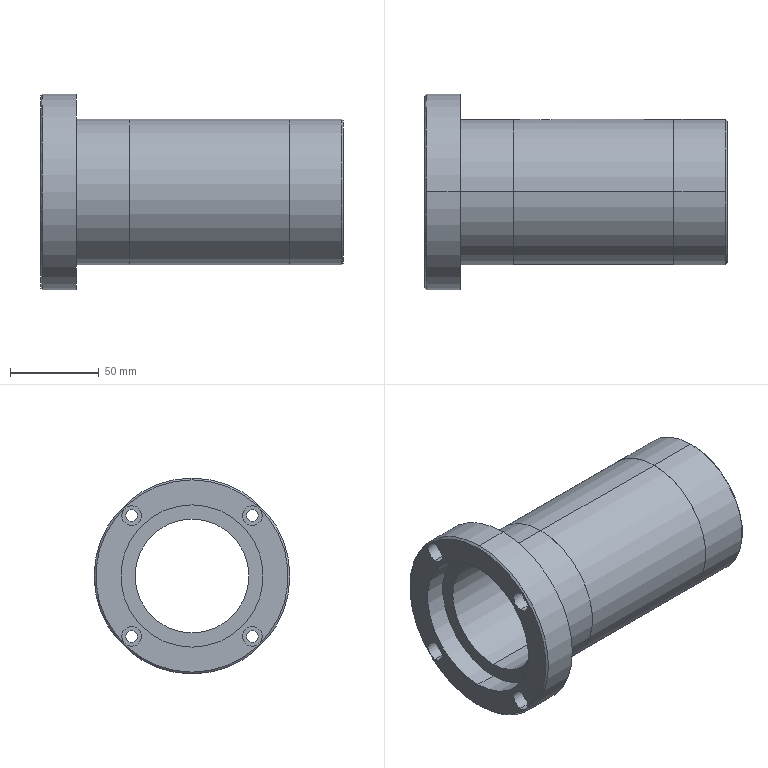Component | SolidWorks | 4-12-12ClampingAxisAssembly-1_4-12-1ClampingTelescopicAxisHousing-1 | 1 solid | 49 faces | box 170 x 110 x 110 mm | volume 405832 mm3 | cylinder 32 | plane 11 | cone 6 | commonest cylinder face diameters 11 x8 6.6 x8 82 x4 10 x2 80 x2 64 x2 81.8 x2 110 x2
build123d program:
from build123d import *

# Parameters (mm, degrees)
HOLE_SIZE_ACCORDING_TO_THE_TYPE_OF_HEX_S_D           = 6.6
HOLE_SIZE_ACCORDING_TO_THE_TYPE_OF_HEX_S_CBORE_D     = 11
HOLE_SIZE_ACCORDING_TO_THE_TYPE_OF_HEX_S_CBORE_DEPTH = 6.8
CIRPATTERN1_COUNT                                    = 4
SKETCH6_W                                            = 4.25
SKETCH6_H                                            = 55
CHAMFER1_SIZE                                        = 1
SKETCH1_R                                            = 5
M10_THREAD_MAJOR_DIAMETER_RELEASE_DEPTH              = 12


with BuildPart() as part:
    # Sketch1_2 → Revolve1 (revolve)
    with BuildSketch(Plane.XY, mode=Mode.PRIVATE) as revolve1_sk:
        Polygon((0, 40), (0, 55), (20, 55), (20, 41), (50, 41), (50, 40.9), (140, 40.9), (140, 41), (170, 41), (170, 32), (12, 32), (12, 40), align=None)
    revolve(revolve1_sk.sketch.rotate(Axis((0, 0, 0), (1, 0, 0)), 90), axis=Axis((0, 0, 0), (1, 0, 0)))

    # Hole Size according to the type of Hex S (through all)
    with Locations(Plane.ZY):
        with Locations((33.941, 33.941)):
            hole_size_according_to_the_type_of_hex_s = CounterBoreHole(HOLE_SIZE_ACCORDING_TO_THE_TYPE_OF_HEX_S_D / 2, HOLE_SIZE_ACCORDING_TO_THE_TYPE_OF_HEX_S_CBORE_D / 2, HOLE_SIZE_ACCORDING_TO_THE_TYPE_OF_HEX_S_CBORE_DEPTH)

    # CirPattern1: Hole Size according to the type of Hex S ×4 about axis
    cirpattern1_axis = Axis((0, 0, 0), (1, 0, 0))
    for i in range(1, CIRPATTERN1_COUNT):
        add(hole_size_according_to_the_type_of_hex_s.rotate(cirpattern1_axis, i * 360 / CIRPATTERN1_COUNT), mode=Mode.SUBTRACT)

    # Sketch6 → M10 Tapped Hole1 (revolve, cut)
    with BuildSketch(Plane(origin=(68, 0, 0), x_dir=(0, 0, -1), z_dir=(1, 0, 0))):
        with Locations((2.125, 27.5)):
            Rectangle(SKETCH6_W, SKETCH6_H)
    revolve(axis=Axis((68, -6.35, 0), (0, 1, 0)), mode=Mode.SUBTRACT)

    # Chamfer1
    chamfer1_edges = [part.edges().sort_by_distance(p)[0] for p in [
        (170, 0, -32),
        (170, 0, -41),
        (0, 0, -55),
    ]]
    chamfer(chamfer1_edges, length=CHAMFER1_SIZE)

    # Sketch1 → M10 Thread Major Diameter Release (cut)
    with BuildSketch(Plane(origin=(0, 45, 0), x_dir=(1, 0, 0), z_dir=(0, 1, 0))):
        with Locations(Location((68, 0, 0), (0, 0, 270))):
            Circle(SKETCH1_R)
    extrude(amount=-M10_THREAD_MAJOR_DIAMETER_RELEASE_DEPTH, mode=Mode.SUBTRACT)


solid = part.part

# Placed as in the assembly
solid = solid.moved(Location((-87.809, -4.181, 0.0001024), (0, 0, 0)))